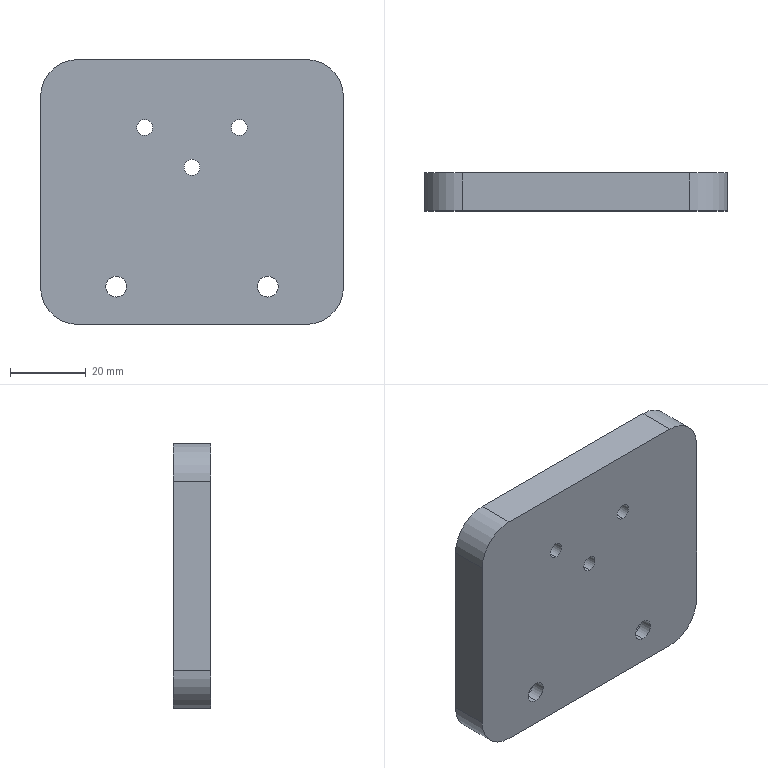CAM job | Mastercam | mm | 8 operations | part box 80 x 10 x 70
1. Facing | 20 - 63 平铣刀
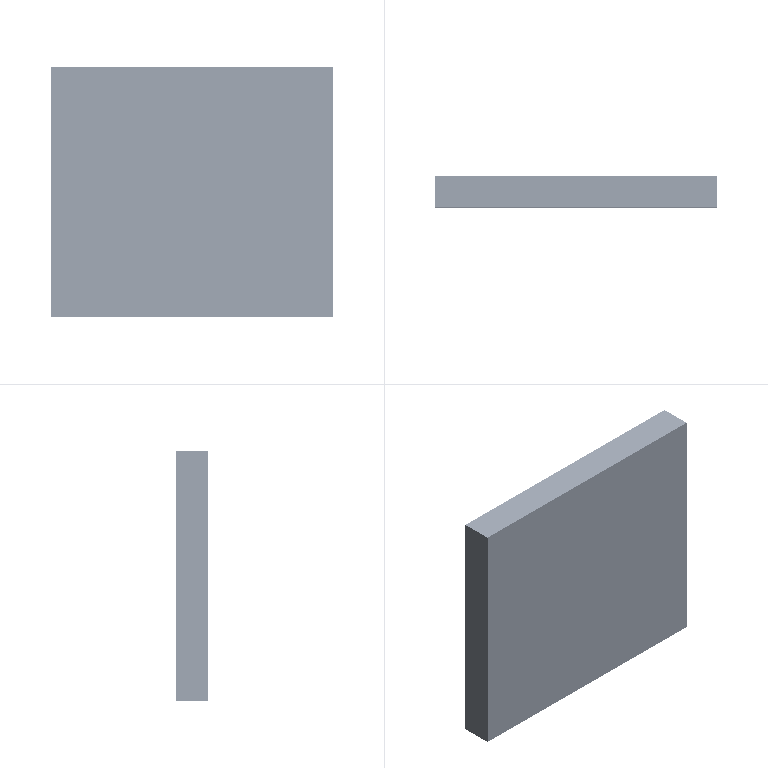2. 2D High Speed (2D Dynamic Mill) | 9 - 10 平铣刀
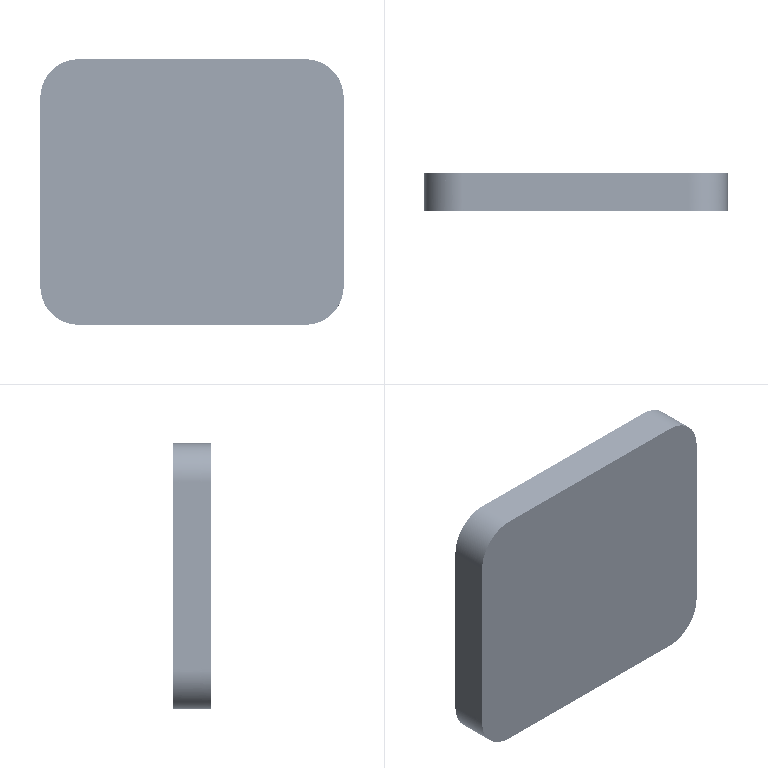3. Contour (2D) | 10 - 10 平铣刀
4. Helix Bore | 6 - 6 平铣刀
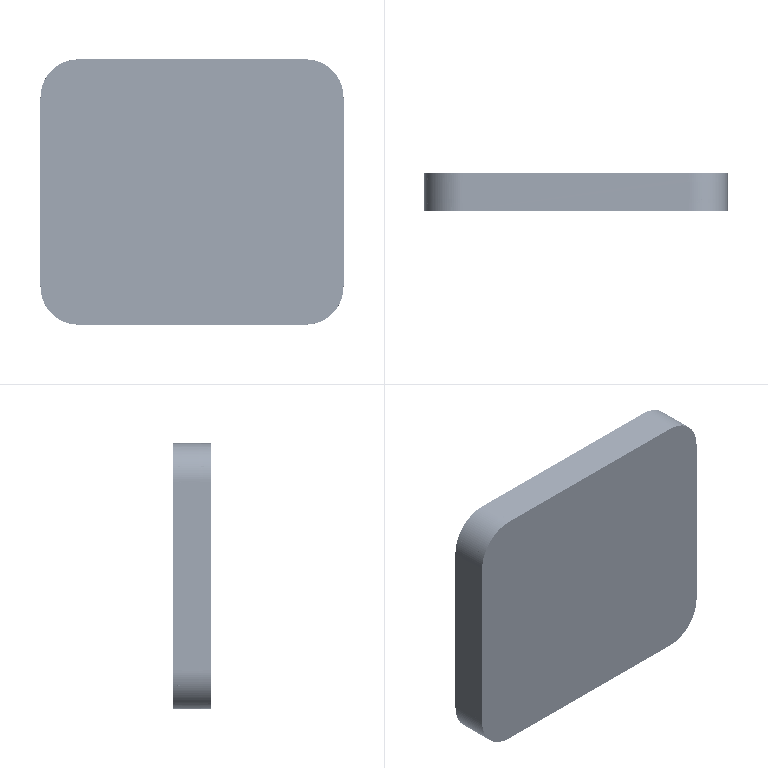5. Drill/Counterbore | 7 - 4 倒角刀
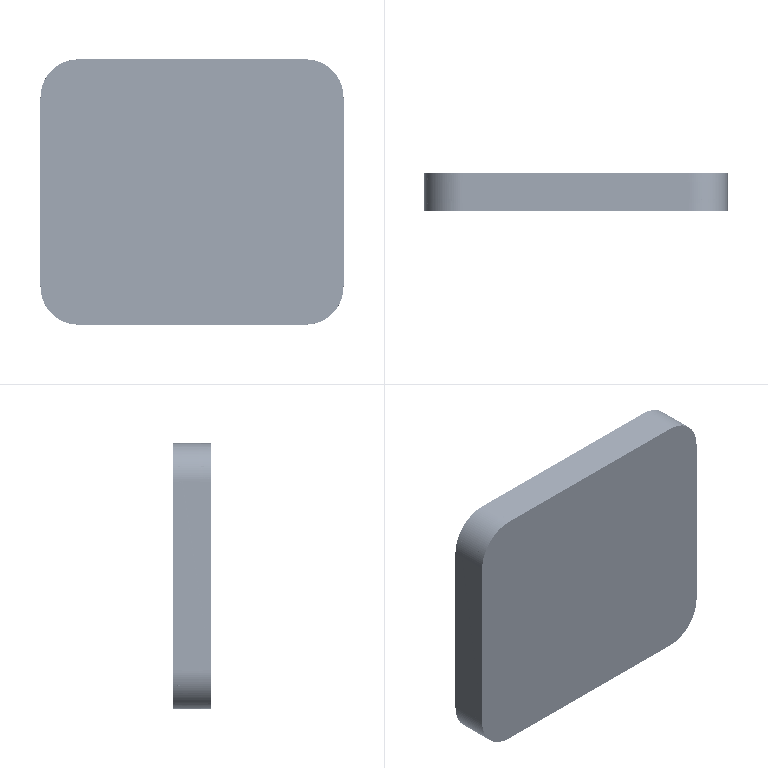6. Contour (2D chamfer) | 7 - 4 倒角刀
7. Facing | 20 - 63 平铣刀
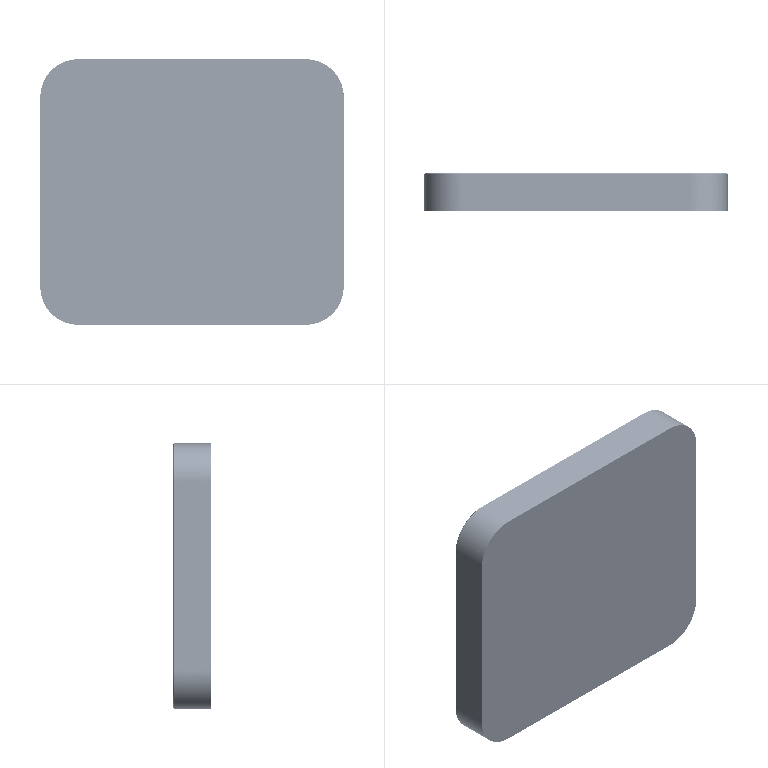8. Contour (2D chamfer) | 7 - 4 倒角刀